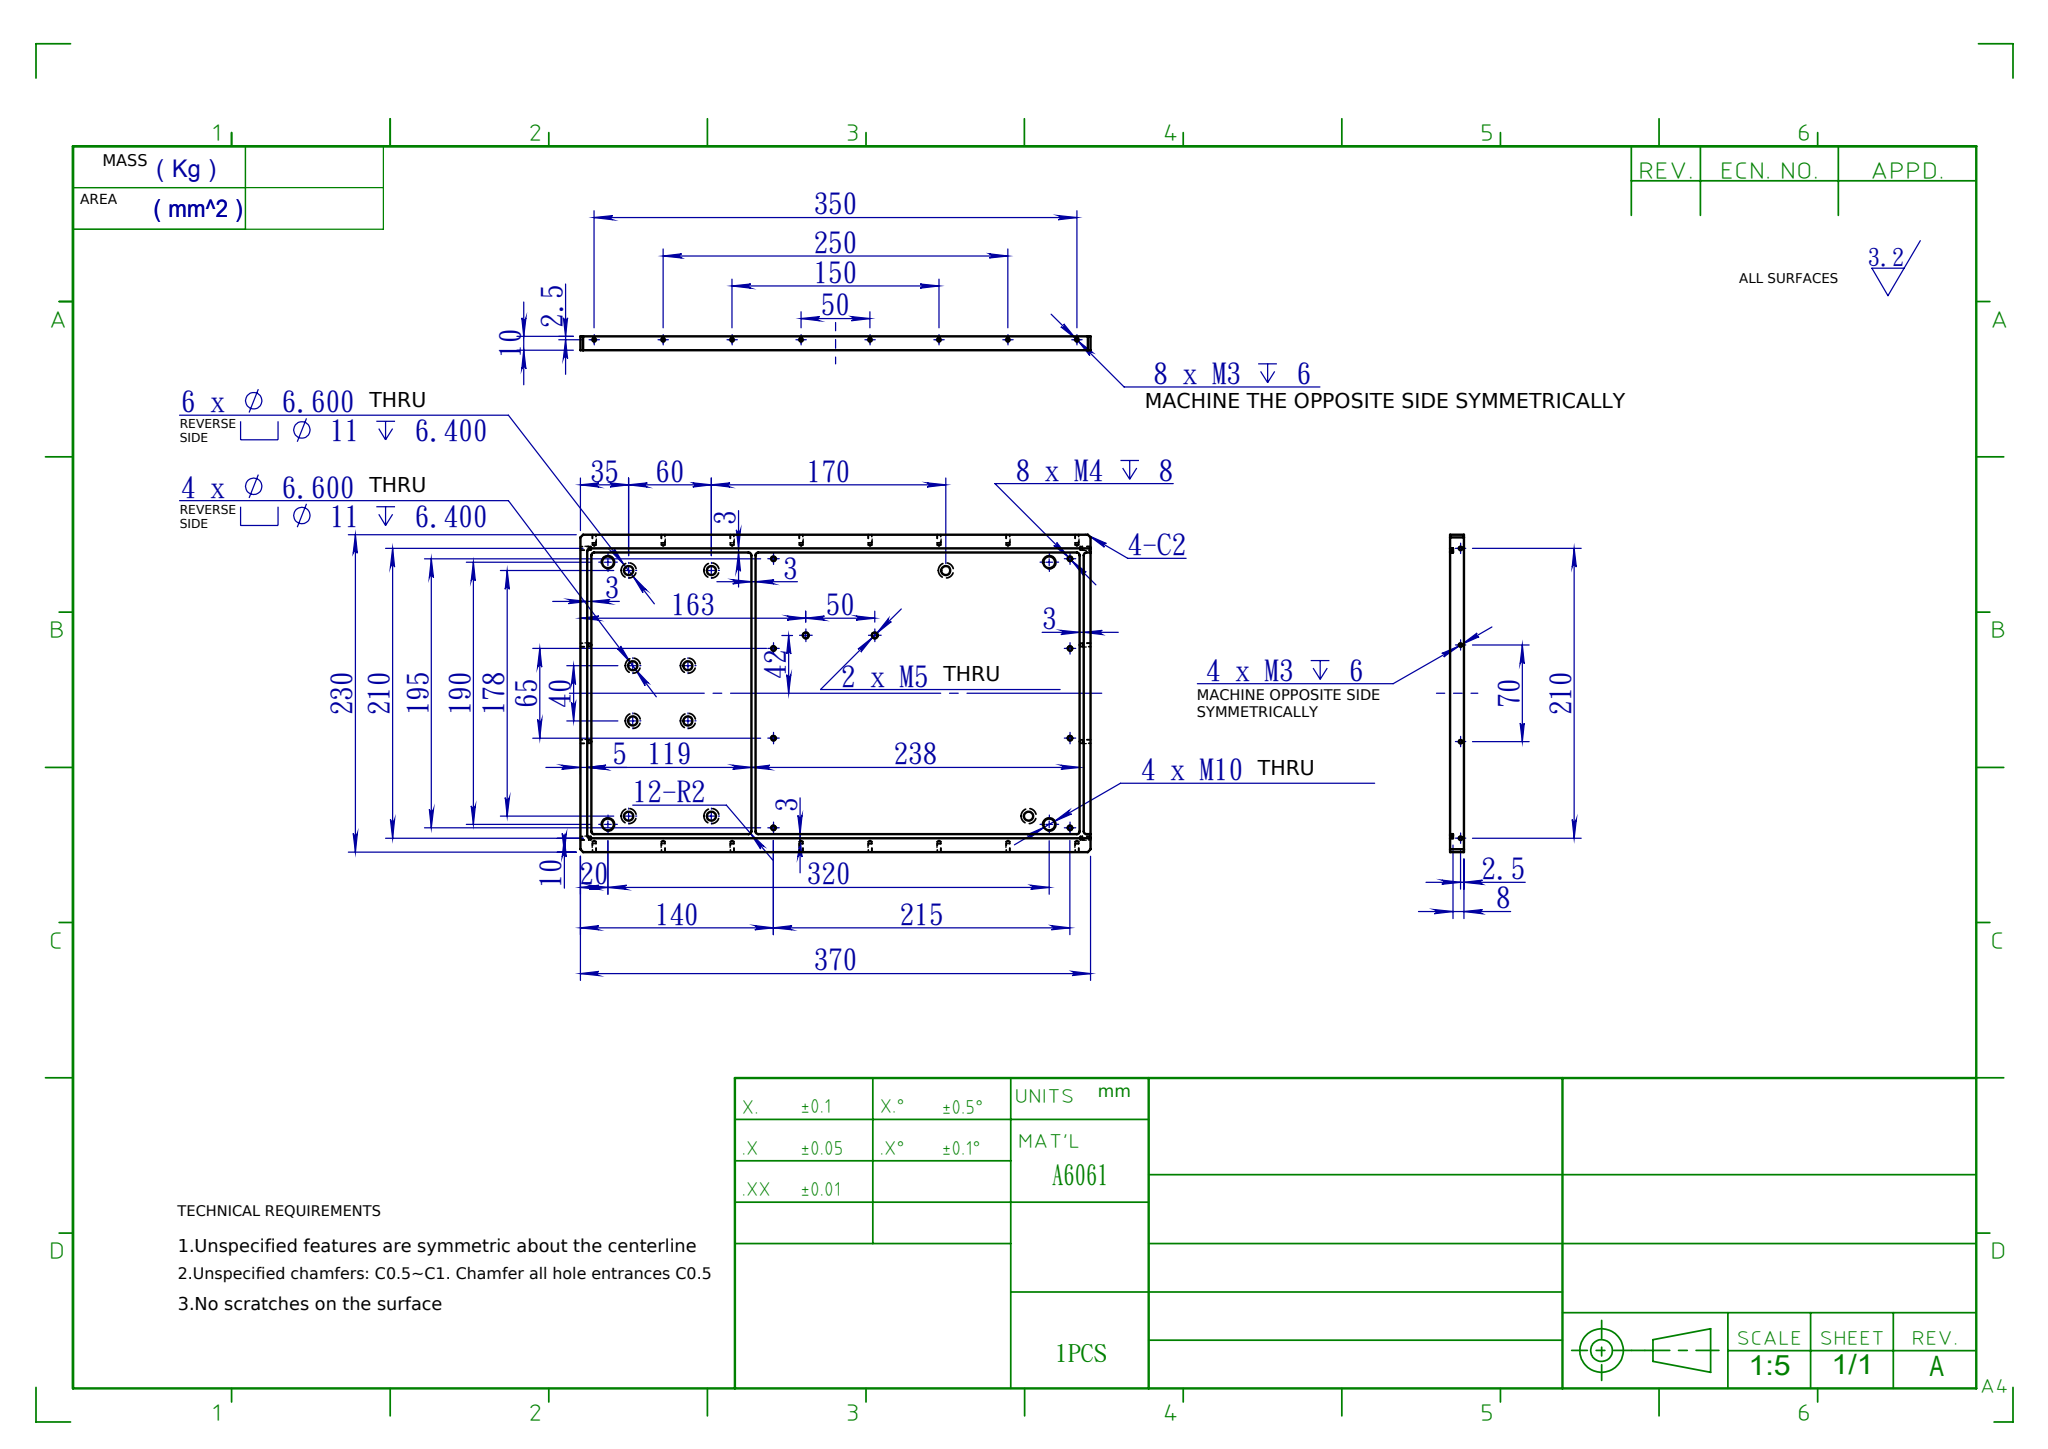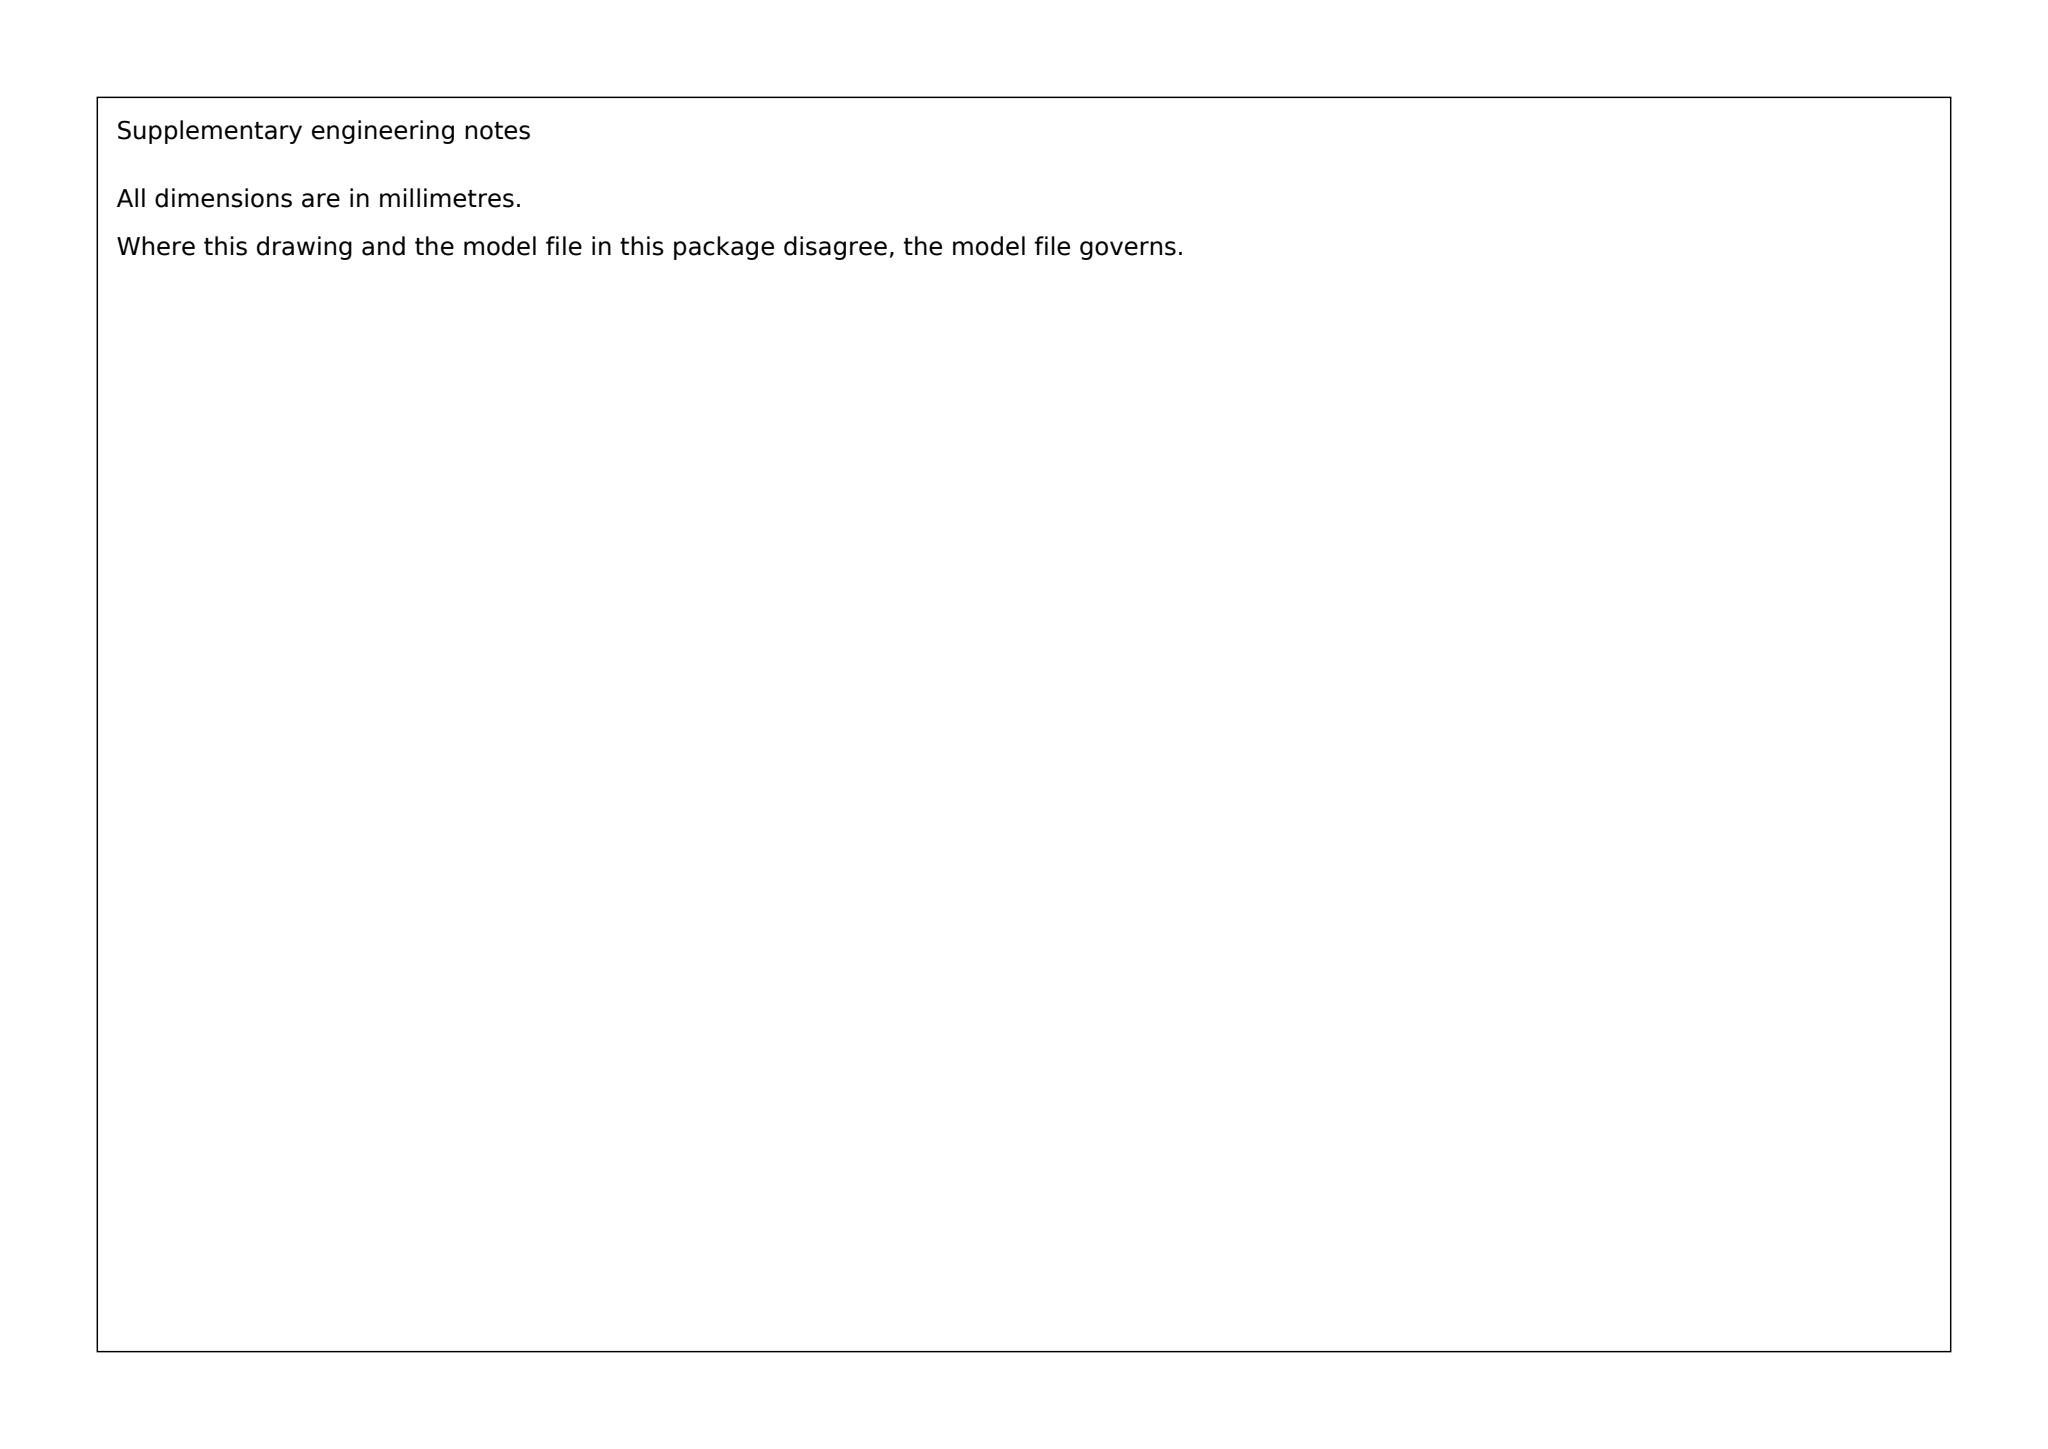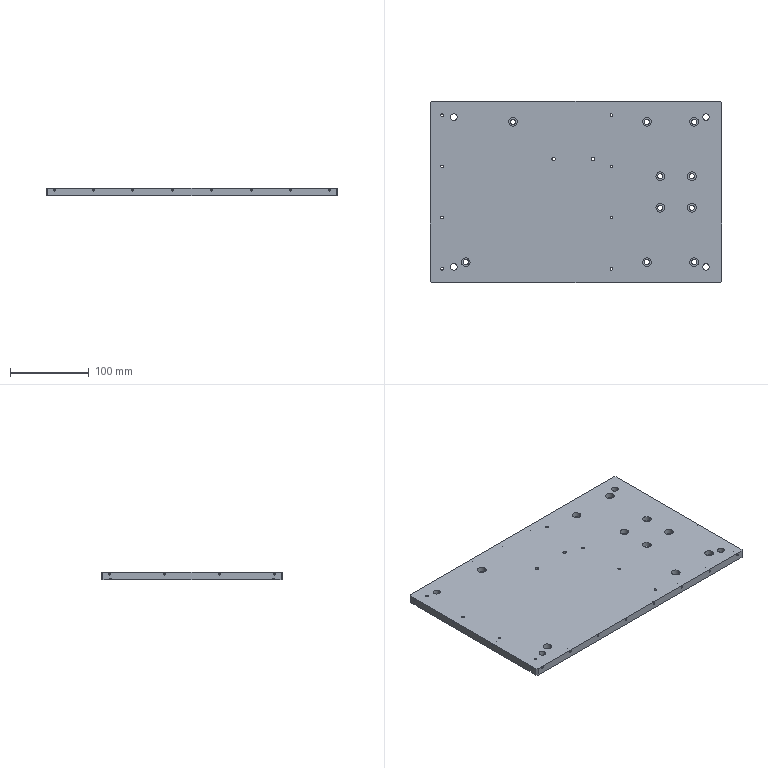Part | SolidWorks | mm | material A6061 | 1 solid | 214 faces | box 370 x 230 x 10 mm | volume 831396 mm3 | cylinder 128 | cone 48 | plane 38 | commonest cylinder face diameters 2.5 x48 11 x20 6.6 x20 3.3 x16 4 x12 8.5 x8 4.2 x4
build123d program:
from build123d import *

# Parameters (mm, degrees)
SKETCH1_2_W                                         = 370
SKETCH1_2_H                                         = 230
BOSS_EXTRUDE1_2_DEPTH                               = 10
CHAMFER1_SIZE                                       = 2
COUNTERBORE_HOLE_FOR_M6_HEX_SOCKET_HEAD_D           = 6.6
COUNTERBORE_HOLE_FOR_M6_HEX_SOCKET_HEAD_CBORE_D     = 11
COUNTERBORE_HOLE_FOR_M6_HEX_SOCKET_HEAD_CBORE_DEPTH = 6.4
CBORE_FOR_M6_HEX_SOCKET_HEAD_CAP_SCREW2_D           = 6.6
CBORE_FOR_M6_HEX_SOCKET_HEAD_CAP_SCREW2_CBORE_D     = 11
CBORE_FOR_M6_HEX_SOCKET_HEAD_CAP_SCREW2_CBORE_DEPTH = 6.4
M3_TAPPED_HOLE1_AT_2_COUNT                          = 2
M3_TAPPED_HOLE1_AT_2_PITCH                          = 50
M3_TAPPED_HOLE1_AT_3_COUNT                          = 2
M3_TAPPED_HOLE1_AT_3_PITCH                          = 100
M3_TAPPED_HOLE1_AT_4_COUNT                          = 2
M3_TAPPED_HOLE1_AT_4_PITCH                          = 150
M3_TAPPED_HOLE1_AT_5_COUNT                          = 2
M3_TAPPED_HOLE1_AT_5_PITCH                          = 200
M3_TAPPED_HOLE1_AT_6_COUNT                          = 2
M3_TAPPED_HOLE1_AT_6_PITCH                          = 250
M3_TAPPED_HOLE1_AT_7_COUNT                          = 2
M3_TAPPED_HOLE1_AT_7_PITCH                          = 300
M3_TAPPED_HOLE1_AT_8_COUNT                          = 2
M3_TAPPED_HOLE1_AT_8_PITCH                          = 350
M3_TAPPED_HOLE2_AT_2_COUNT                          = 2
M3_TAPPED_HOLE2_AT_2_PITCH                          = 70
M3_TAPPED_HOLE2_AT_3_COUNT                          = 2
M3_TAPPED_HOLE2_AT_3_PITCH                          = 140
M3_TAPPED_HOLE2_AT_4_COUNT                          = 2
M3_TAPPED_HOLE2_AT_4_PITCH                          = 210
M10_TAPPED_HOLE1_D                                  = 8.5
SKETCH13_W                                          = 370
SKETCH13_H                                          = 3
CUT_EXTRUDE1_DEPTH                                  = 2
SKETCH14_W                                          = 3
SKETCH14_H                                          = 204
CUT_EXTRUDE2_DEPTH                                  = 2
SKETCH15_W                                          = 5
SKETCH15_H                                          = 3
BOSS_EXTRUDE1_DEPTH                                 = 2
FILLET1_R                                           = 2
M5_TAPPED_HOLE1_D                                   = 4.2
M4_TAPPED_HOLE1_D                                   = 3.3
M4_TAPPED_HOLE1_DEPTH                               = 10.1
M4_TAPPED_HOLE1_TIP                                 = 0.9914


with BuildPart() as part:
    # Sketch1_2 → Boss-Extrude1_2 (new body)
    with BuildSketch(Plane.XY):
        Rectangle(SKETCH1_2_W, SKETCH1_2_H)
    extrude(amount=BOSS_EXTRUDE1_2_DEPTH)

    # Chamfer1
    chamfer1_edges = [part.edges().sort_by_distance(p)[0] for p in [
        (-185, 115, 5),
        (185, 115, 5),
        (185, -115, 5),
        (-185, -115, 5),
    ]]
    chamfer(chamfer1_edges, length=CHAMFER1_SIZE)

    # Counterbore Hole for M6 Hex Socket Head (through all)
    with Locations(Plane.XY.offset(10)):
        with Locations((90, 89), (150, 89), (90, -89), (150, -89), (-80, 89), (-140, -89)):
            CounterBoreHole(COUNTERBORE_HOLE_FOR_M6_HEX_SOCKET_HEAD_D / 2, COUNTERBORE_HOLE_FOR_M6_HEX_SOCKET_HEAD_CBORE_D / 2, COUNTERBORE_HOLE_FOR_M6_HEX_SOCKET_HEAD_CBORE_DEPTH)

    # CBORE for M6 Hex Socket Head Cap Screw2 (through all)
    with Locations(Plane.XY.offset(10)):
        with Locations((107, 20), (107, -20), (147, -20), (147, 20)):
            CounterBoreHole(CBORE_FOR_M6_HEX_SOCKET_HEAD_CAP_SCREW2_D / 2, CBORE_FOR_M6_HEX_SOCKET_HEAD_CAP_SCREW2_CBORE_D / 2, CBORE_FOR_M6_HEX_SOCKET_HEAD_CAP_SCREW2_CBORE_DEPTH)

    # Sketch7 → M3 Tapped Hole1 (revolve, cut)
    with BuildSketch(Plane(origin=(175, -115, 7.5), x_dir=(0, 0, -1), z_dir=(1, 0, 0))):
        Polygon((0, 0), (0, 8.251), (1.25, 7.5), (1.25, 0), align=None)
    m3_tapped_hole1 = revolve(axis=Axis((175, -121.35, 7.5), (0, 1, 0)), mode=Mode.SUBTRACT)

    # M3 Tapped Hole1 at 2: M3 Tapped Hole1 ×2
    with Locations(*[(-i * M3_TAPPED_HOLE1_AT_2_PITCH, 0, 0) for i in range(1, M3_TAPPED_HOLE1_AT_2_COUNT)]):
        add(m3_tapped_hole1, mode=Mode.SUBTRACT)

    # M3 Tapped Hole1 at 3: M3 Tapped Hole1 ×2
    with Locations(*[(-i * M3_TAPPED_HOLE1_AT_3_PITCH, 0, 0) for i in range(1, M3_TAPPED_HOLE1_AT_3_COUNT)]):
        add(m3_tapped_hole1, mode=Mode.SUBTRACT)

    # M3 Tapped Hole1 at 4: M3 Tapped Hole1 ×2
    with Locations(*[(-i * M3_TAPPED_HOLE1_AT_4_PITCH, 0, 0) for i in range(1, M3_TAPPED_HOLE1_AT_4_COUNT)]):
        add(m3_tapped_hole1, mode=Mode.SUBTRACT)

    # M3 Tapped Hole1 at 5: M3 Tapped Hole1 ×2
    with Locations(*[(-i * M3_TAPPED_HOLE1_AT_5_PITCH, 0, 0) for i in range(1, M3_TAPPED_HOLE1_AT_5_COUNT)]):
        add(m3_tapped_hole1, mode=Mode.SUBTRACT)

    # M3 Tapped Hole1 at 6: M3 Tapped Hole1 ×2
    with Locations(*[(-i * M3_TAPPED_HOLE1_AT_6_PITCH, 0, 0) for i in range(1, M3_TAPPED_HOLE1_AT_6_COUNT)]):
        add(m3_tapped_hole1, mode=Mode.SUBTRACT)

    # M3 Tapped Hole1 at 7: M3 Tapped Hole1 ×2
    with Locations(*[(-i * M3_TAPPED_HOLE1_AT_7_PITCH, 0, 0) for i in range(1, M3_TAPPED_HOLE1_AT_7_COUNT)]):
        add(m3_tapped_hole1, mode=Mode.SUBTRACT)

    # M3 Tapped Hole1 at 8: M3 Tapped Hole1 ×2
    with Locations(*[(-i * M3_TAPPED_HOLE1_AT_8_PITCH, 0, 0) for i in range(1, M3_TAPPED_HOLE1_AT_8_COUNT)]):
        add(m3_tapped_hole1, mode=Mode.SUBTRACT)

    # Mirror1: M3 Tapped Hole1 across plane
    add(m3_tapped_hole1.mirror(Plane.ZX), mode=Mode.SUBTRACT)

    # Mirror1 copy 1 sketch → Mirror1 copy 1 (revolve, cut)
    with BuildSketch(Plane(origin=(125, 115, 7.5), x_dir=(0, 0, -1), z_dir=(1, 0, 0))):
        Polygon((0, 0), (0, -8.251), (1.25, -7.5), (1.25, 0), align=None)
    revolve(axis=Axis((125, 121.35, 7.5), (0, 1, 0)), mode=Mode.SUBTRACT)

    # Mirror1 copy 2 sketch → Mirror1 copy 2 (revolve, cut)
    with BuildSketch(Plane(origin=(75, 115, 7.5), x_dir=(0, 0, -1), z_dir=(1, 0, 0))):
        Polygon((0, 0), (0, -8.251), (1.25, -7.5), (1.25, 0), align=None)
    revolve(axis=Axis((75, 121.35, 7.5), (0, 1, 0)), mode=Mode.SUBTRACT)

    # Mirror1 copy 3 sketch → Mirror1 copy 3 (revolve, cut)
    with BuildSketch(Plane(origin=(25, 115, 7.5), x_dir=(0, 0, -1), z_dir=(1, 0, 0))):
        Polygon((0, 0), (0, -8.251), (1.25, -7.5), (1.25, 0), align=None)
    revolve(axis=Axis((25, 121.35, 7.5), (0, 1, 0)), mode=Mode.SUBTRACT)

    # Mirror1 copy 4 sketch → Mirror1 copy 4 (revolve, cut)
    with BuildSketch(Plane(origin=(-25, 115, 7.5), x_dir=(0, 0, -1), z_dir=(1, 0, 0))):
        Polygon((0, 0), (0, -8.251), (1.25, -7.5), (1.25, 0), align=None)
    revolve(axis=Axis((-25, 121.35, 7.5), (0, 1, 0)), mode=Mode.SUBTRACT)

    # Mirror1 copy 5 sketch → Mirror1 copy 5 (revolve, cut)
    with BuildSketch(Plane(origin=(-75, 115, 7.5), x_dir=(0, 0, -1), z_dir=(1, 0, 0))):
        Polygon((0, 0), (0, -8.251), (1.25, -7.5), (1.25, 0), align=None)
    revolve(axis=Axis((-75, 121.35, 7.5), (0, 1, 0)), mode=Mode.SUBTRACT)

    # Mirror1 copy 6 sketch → Mirror1 copy 6 (revolve, cut)
    with BuildSketch(Plane(origin=(-125, 115, 7.5), x_dir=(0, 0, -1), z_dir=(1, 0, 0))):
        Polygon((0, 0), (0, -8.251), (1.25, -7.5), (1.25, 0), align=None)
    revolve(axis=Axis((-125, 121.35, 7.5), (0, 1, 0)), mode=Mode.SUBTRACT)

    # Mirror1 copy 7 sketch → Mirror1 copy 7 (revolve, cut)
    with BuildSketch(Plane(origin=(-175, 115, 7.5), x_dir=(0, 0, -1), z_dir=(1, 0, 0))):
        Polygon((0, 0), (0, -8.251), (1.25, -7.5), (1.25, 0), align=None)
    revolve(axis=Axis((-175, 121.35, 7.5), (0, 1, 0)), mode=Mode.SUBTRACT)

    # Sketch9 → M3 Tapped Hole2 (revolve, cut)
    with BuildSketch(Plane(origin=(185, 105, 7.5), x_dir=(0, 0, -1), z_dir=(0, 1, 0))):
        Polygon((0, 0), (0, 8.251), (1.25, 7.5), (1.25, 0), align=None)
    m3_tapped_hole2 = revolve(axis=Axis((191.35, 105, 7.5), (-1, 0, 0)), mode=Mode.SUBTRACT)

    # M3 Tapped Hole2 at 2: M3 Tapped Hole2 ×2
    with Locations(*[(0, -i * M3_TAPPED_HOLE2_AT_2_PITCH, 0) for i in range(1, M3_TAPPED_HOLE2_AT_2_COUNT)]):
        add(m3_tapped_hole2, mode=Mode.SUBTRACT)

    # M3 Tapped Hole2 at 3: M3 Tapped Hole2 ×2
    with Locations(*[(0, -i * M3_TAPPED_HOLE2_AT_3_PITCH, 0) for i in range(1, M3_TAPPED_HOLE2_AT_3_COUNT)]):
        add(m3_tapped_hole2, mode=Mode.SUBTRACT)

    # M3 Tapped Hole2 at 4: M3 Tapped Hole2 ×2
    with Locations(*[(0, -i * M3_TAPPED_HOLE2_AT_4_PITCH, 0) for i in range(1, M3_TAPPED_HOLE2_AT_4_COUNT)]):
        add(m3_tapped_hole2, mode=Mode.SUBTRACT)

    # Mirror2: M3 Tapped Hole2 across plane
    add(m3_tapped_hole2.mirror(Plane(origin=(0, 0, 0), x_dir=(0, 0, 1), z_dir=(1, 0, 0))), mode=Mode.SUBTRACT)

    # Mirror2 copy 1 sketch → Mirror2 copy 1 (revolve, cut)
    with BuildSketch(Plane(origin=(-185, 35, 7.5), x_dir=(0, 0, -1), z_dir=(0, 1, 0))):
        Polygon((0, 0), (0, -8.251), (1.25, -7.5), (1.25, 0), align=None)
    revolve(axis=Axis((-191.35, 35, 7.5), (-1, 0, 0)), mode=Mode.SUBTRACT)

    # Mirror2 copy 2 sketch → Mirror2 copy 2 (revolve, cut)
    with BuildSketch(Plane(origin=(-185, -35, 7.5), x_dir=(0, 0, -1), z_dir=(0, 1, 0))):
        Polygon((0, 0), (0, -8.251), (1.25, -7.5), (1.25, 0), align=None)
    revolve(axis=Axis((-191.35, -35, 7.5), (-1, 0, 0)), mode=Mode.SUBTRACT)

    # Mirror2 copy 3 sketch → Mirror2 copy 3 (revolve, cut)
    with BuildSketch(Plane(origin=(-185, -105, 7.5), x_dir=(0, 0, -1), z_dir=(0, 1, 0))):
        Polygon((0, 0), (0, -8.251), (1.25, -7.5), (1.25, 0), align=None)
    revolve(axis=Axis((-191.35, -105, 7.5), (-1, 0, 0)), mode=Mode.SUBTRACT)

    # M10 Tapped Hole1 (through all)
    with Locations(Plane.XY.offset(10)):
        with Locations((-155, 95), (-155, -95), (165, 95), (165, -95)):
            Hole(M10_TAPPED_HOLE1_D / 2)

    # Sketch13 → Cut-Extrude1 (cut)
    with BuildSketch(Plane(origin=(0, 0, 0), x_dir=(-1, 0, 0), z_dir=(0, 0, -1))):
        with Locations((0, 103.5)):
            Rectangle(SKETCH13_W, SKETCH13_H)
        with Locations((0, -103.5)):
            Rectangle(SKETCH13_W, SKETCH13_H)
    extrude(amount=-CUT_EXTRUDE1_DEPTH, mode=Mode.SUBTRACT)

    # Sketch14 → Cut-Extrude2 (cut)
    with BuildSketch(Plane(origin=(0, 0, 0), x_dir=(-1, 0, 0), z_dir=(0, 0, -1))):
        with Locations((-59.5, 0)):
            Rectangle(SKETCH14_W, SKETCH14_H)
        with Locations((178.5, 0)):
            Rectangle(SKETCH14_W, SKETCH14_H)
        with Locations((-178.5, 0)):
            Rectangle(SKETCH14_W, SKETCH14_H)
    extrude(amount=-CUT_EXTRUDE2_DEPTH, mode=Mode.SUBTRACT)

    # Sketch15 → Boss-Extrude1 (add)
    with BuildSketch(Plane(origin=(0, 0, 2), x_dir=(-1, 0, 0), z_dir=(0, 0, -1))):
        with Locations((-182.5, 103.5)):
            Rectangle(SKETCH15_W, SKETCH15_H)
        with Locations((-182.5, -103.5)):
            Rectangle(SKETCH15_W, SKETCH15_H)
    extrude(amount=BOSS_EXTRUDE1_DEPTH)

    # Fillet1
    fillet1_edges = [part.edges().sort_by_distance(p)[0] for p in [
        (61, -102, 1),
        (61, 102, 1),
        (58, 102, 1),
        (58, -102, 1),
        (-180, 102, 1),
        (-180, -102, 1),
        (-177, -102, 1),
        (-177, 102, 1),
        (177, 102, 1),
        (177, -102, 1),
        (180, 105, 1),
        (180, -105, 1),
    ]]
    fillet(fillet1_edges, radius=FILLET1_R)

    # M5 Tapped Hole1 (through all)
    with Locations(Plane(origin=(0, 0, 0), x_dir=(-1, 0, 0), z_dir=(0, 0, -1))):
        with Locations((28.46, 42), (-21.54, 42)):
            Hole(M5_TAPPED_HOLE1_D / 2)

    # M4 Tapped Hole1
    with Locations(Plane(origin=(0, 0, 0), x_dir=(-1, 0, 0), z_dir=(0, 0, -1))):
        with Locations((-45, 97.5), (-45, 32.5), (-45, -32.5), (-45, -97.5), (170, 97.5), (170, 32.5), (170, -32.5), (170, -97.5)):
            Hole(M4_TAPPED_HOLE1_D / 2, depth=M4_TAPPED_HOLE1_DEPTH)
            with Locations((0, 0, -(M4_TAPPED_HOLE1_DEPTH + M4_TAPPED_HOLE1_TIP / 2))):  # 118° drill point
                Cone(0, M4_TAPPED_HOLE1_D / 2, M4_TAPPED_HOLE1_TIP, mode=Mode.SUBTRACT)


solid = part.part